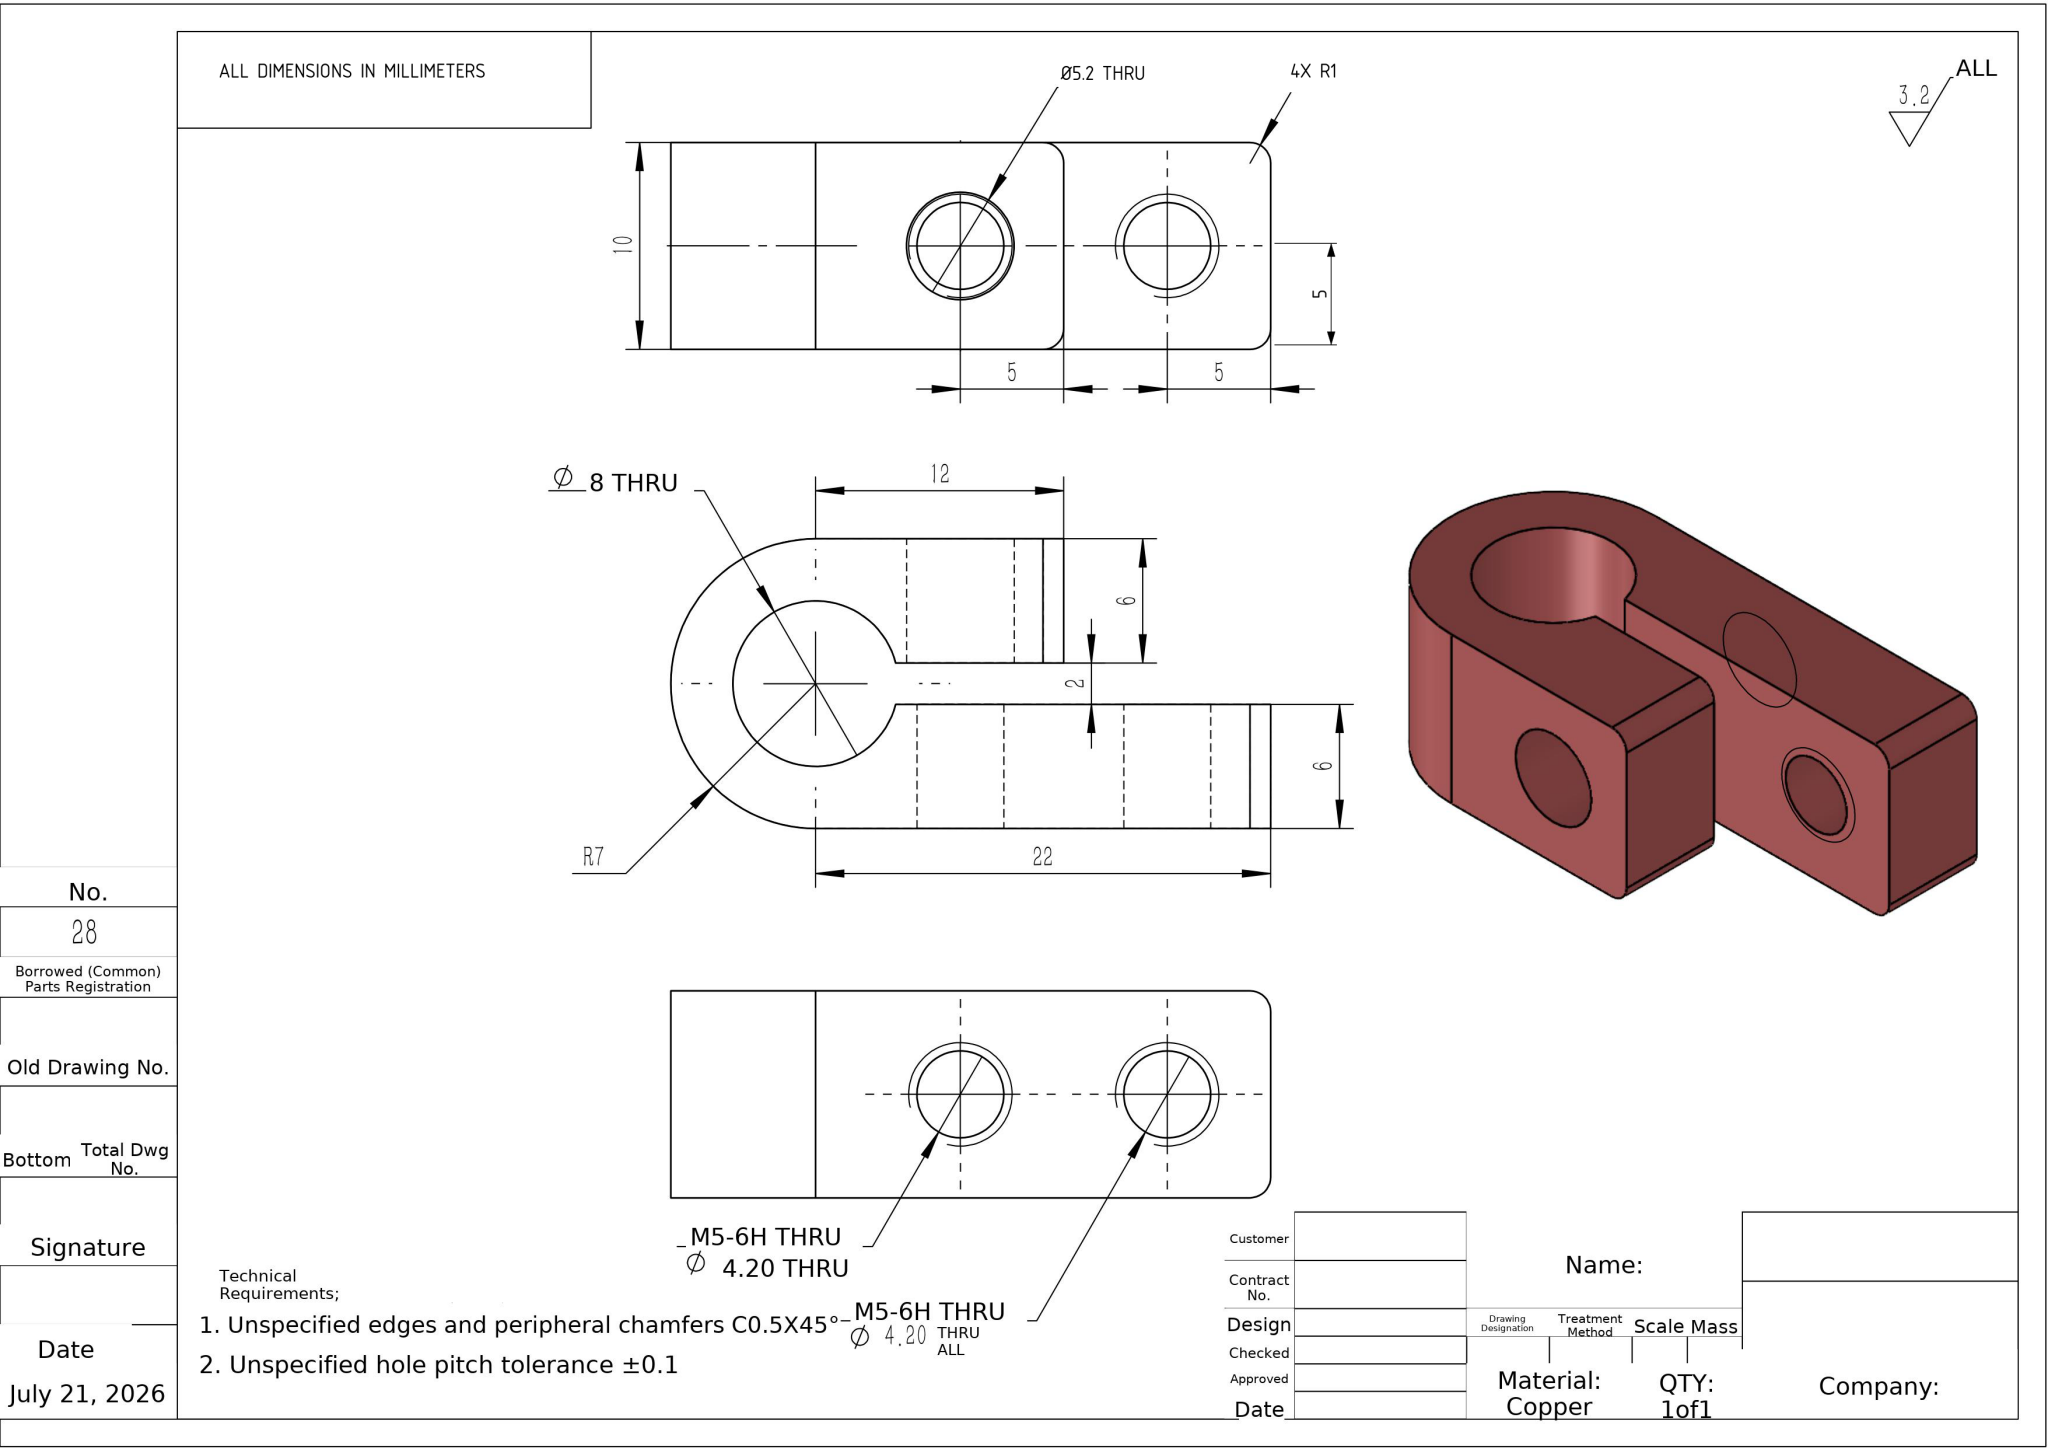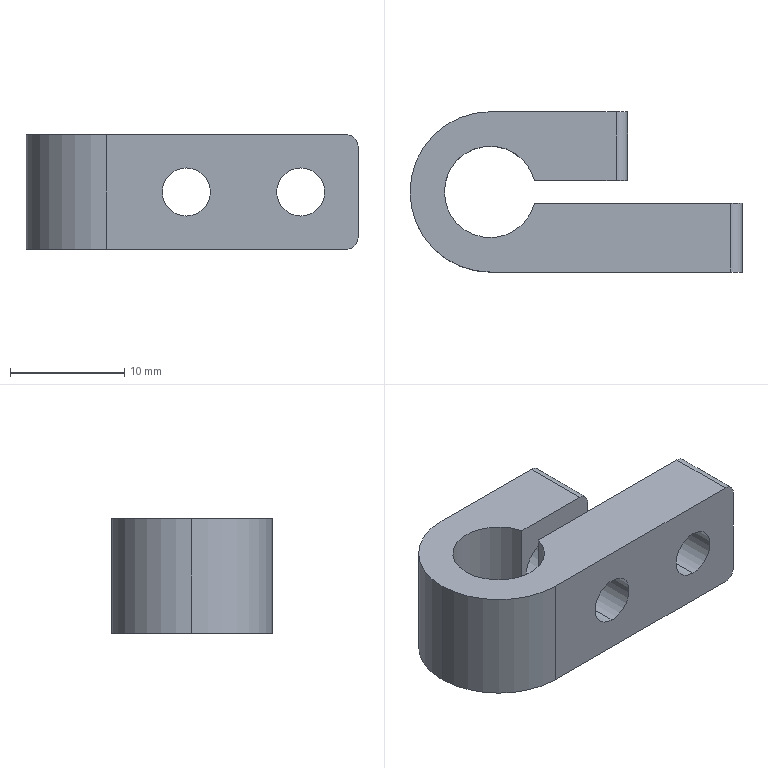Part | NX | mm | Stepped Clevis Bracket | 1 solid | 21 faces | box 29 x 14 x 10 mm | volume 2087 mm3 | cylinder 13 | plane 8 | commonest cylinder face diameters 4.2 x4 2 x4 5.2 x2 14 x2 8 x1
STEP:
#1=COLOUR_RGB('',0.7922,0.8196,0.9333);
#2=FILL_AREA_STYLE_COLOUR('',#1);
#3=FILL_AREA_STYLE('',(#2));
#4=SURFACE_STYLE_FILL_AREA(#3);
#5=SURFACE_SIDE_STYLE('',(#4));
#6=SURFACE_STYLE_USAGE(.BOTH.,#5);
#7=PRESENTATION_STYLE_ASSIGNMENT((#6));
#8=CARTESIAN_POINT('',(-4.,-1.,7.1));
#9=VERTEX_POINT('',#8);
#10=CARTESIAN_POINT('',(-4.,-1.,2.9));
#11=VERTEX_POINT('',#10);
#12=CARTESIAN_POINT('',(-4.,-1.,5.));
#13=DIRECTION('',(0.,-1.,0.));
#14=DIRECTION('',(1.,0.,0.));
#15=AXIS2_PLACEMENT_3D('',#12,#13,#14);
#16=CIRCLE('',#15,2.1);
#17=EDGE_CURVE('',#9,#11,#16,.T.);
#18=ORIENTED_EDGE('',*,*,#17,.F.);
#19=CARTESIAN_POINT('',(-4.,-7.,7.1));
#20=VERTEX_POINT('',#19);
#21=CARTESIAN_POINT('',(-4.,-7.,7.1));
#22=DIRECTION('',(0.,-1.,0.));
#23=VECTOR('',#22,1000.);
#24=LINE('',#21,#23);
#25=EDGE_CURVE('',#9,#20,#24,.T.);
#26=ORIENTED_EDGE('',*,*,#25,.T.);
#27=CARTESIAN_POINT('',(-4.,-7.,2.9));
#28=VERTEX_POINT('',#27);
#29=CARTESIAN_POINT('',(-4.,-7.,5.));
#30=DIRECTION('',(0.,-1.,0.));
#31=DIRECTION('',(0.,0.,-1.));
#32=AXIS2_PLACEMENT_3D('',#29,#30,#31);
#33=CIRCLE('',#32,2.1);
#34=EDGE_CURVE('',#20,#28,#33,.T.);
#35=ORIENTED_EDGE('',*,*,#34,.T.);
#36=CARTESIAN_POINT('',(-4.,-7.,2.9));
#37=DIRECTION('',(0.,-1.,0.));
#38=VECTOR('',#37,1000.);
#39=LINE('',#36,#38);
#40=EDGE_CURVE('',#11,#28,#39,.T.);
#41=ORIENTED_EDGE('',*,*,#40,.F.);
#42=EDGE_LOOP('',(#18,#26,#35,#41));
#43=FACE_OUTER_BOUND('',#42,.T.);
#44=CARTESIAN_POINT('',(-4.,-7.,5.));
#45=DIRECTION('',(0.,-1.,0.));
#46=DIRECTION('',(0.,0.,-1.));
#47=AXIS2_PLACEMENT_3D('',#44,#45,#46);
#48=CYLINDRICAL_SURFACE('',#47,2.1);
#49=ADVANCED_FACE('',(#43),#48,.F.);
#50=CARTESIAN_POINT('',(-4.,1.,2.4));
#51=VERTEX_POINT('',#50);
#52=CARTESIAN_POINT('',(-4.,1.,7.6));
#53=VERTEX_POINT('',#52);
#54=CARTESIAN_POINT('',(-4.,1.,5.));
#55=DIRECTION('',(-0.,1.,0.));
#56=DIRECTION('',(-1.,-0.,0.));
#57=AXIS2_PLACEMENT_3D('',#54,#55,#56);
#58=CIRCLE('',#57,2.6);
#59=EDGE_CURVE('',#51,#53,#58,.T.);
#60=ORIENTED_EDGE('',*,*,#59,.F.);
#61=CARTESIAN_POINT('',(-4.,7.,2.4));
#62=VERTEX_POINT('',#61);
#63=CARTESIAN_POINT('',(-4.,7.,2.4));
#64=DIRECTION('',(0.,1.,0.));
#65=VECTOR('',#64,1000.);
#66=LINE('',#63,#65);
#67=EDGE_CURVE('',#51,#62,#66,.T.);
#68=ORIENTED_EDGE('',*,*,#67,.T.);
#69=CARTESIAN_POINT('',(-4.,7.,7.6));
#70=VERTEX_POINT('',#69);
#71=CARTESIAN_POINT('',(-4.,7.,5.));
#72=DIRECTION('',(0.,1.,0.));
#73=DIRECTION('',(0.,0.,1.));
#74=AXIS2_PLACEMENT_3D('',#71,#72,#73);
#75=CIRCLE('',#74,2.6);
#76=EDGE_CURVE('',#62,#70,#75,.T.);
#77=ORIENTED_EDGE('',*,*,#76,.T.);
#78=CARTESIAN_POINT('',(-4.,7.,7.6));
#79=DIRECTION('',(0.,1.,0.));
#80=VECTOR('',#79,1000.);
#81=LINE('',#78,#80);
#82=EDGE_CURVE('',#53,#70,#81,.T.);
#83=ORIENTED_EDGE('',*,*,#82,.F.);
#84=EDGE_LOOP('',(#60,#68,#77,#83));
#85=FACE_OUTER_BOUND('',#84,.T.);
#86=CARTESIAN_POINT('',(-4.,7.,5.));
#87=DIRECTION('',(0.,1.,0.));
#88=DIRECTION('',(0.,0.,1.));
#89=AXIS2_PLACEMENT_3D('',#86,#87,#88);
#90=CYLINDRICAL_SURFACE('',#89,2.6);
#91=ADVANCED_FACE('',(#85),#90,.F.);
#92=CARTESIAN_POINT('',(6.,-7.,2.9));
#93=VERTEX_POINT('',#92);
#94=CARTESIAN_POINT('',(6.,-7.,7.1));
#95=VERTEX_POINT('',#94);
#96=CARTESIAN_POINT('',(6.,-7.,5.));
#97=DIRECTION('',(0.,1.,0.));
#98=DIRECTION('',(0.,0.,1.));
#99=AXIS2_PLACEMENT_3D('',#96,#97,#98);
#100=CIRCLE('',#99,2.1);
#101=EDGE_CURVE('',#93,#95,#100,.T.);
#102=ORIENTED_EDGE('',*,*,#101,.F.);
#103=CARTESIAN_POINT('',(6.,-1.,2.9));
#104=VERTEX_POINT('',#103);
#105=CARTESIAN_POINT('',(6.,-1.,2.9));
#106=DIRECTION('',(0.,1.,0.));
#107=VECTOR('',#106,1000.);
#108=LINE('',#105,#107);
#109=EDGE_CURVE('',#93,#104,#108,.T.);
#110=ORIENTED_EDGE('',*,*,#109,.T.);
#111=CARTESIAN_POINT('',(6.,-1.,7.1));
#112=VERTEX_POINT('',#111);
#113=CARTESIAN_POINT('',(6.,-1.,5.));
#114=DIRECTION('',(0.,1.,0.));
#115=DIRECTION('',(0.,0.,1.));
#116=AXIS2_PLACEMENT_3D('',#113,#114,#115);
#117=CIRCLE('',#116,2.1);
#118=EDGE_CURVE('',#104,#112,#117,.T.);
#119=ORIENTED_EDGE('',*,*,#118,.T.);
#120=CARTESIAN_POINT('',(6.,-1.,7.1));
#121=DIRECTION('',(0.,1.,0.));
#122=VECTOR('',#121,1000.);
#123=LINE('',#120,#122);
#124=EDGE_CURVE('',#95,#112,#123,.T.);
#125=ORIENTED_EDGE('',*,*,#124,.F.);
#126=EDGE_LOOP('',(#102,#110,#119,#125));
#127=FACE_OUTER_BOUND('',#126,.T.);
#128=CARTESIAN_POINT('',(6.,-1.,5.));
#129=DIRECTION('',(0.,1.,0.));
#130=DIRECTION('',(0.,0.,1.));
#131=AXIS2_PLACEMENT_3D('',#128,#129,#130);
#132=CYLINDRICAL_SURFACE('',#131,2.1);
#133=ADVANCED_FACE('',(#127),#132,.F.);
#134=CARTESIAN_POINT('',(-18.,-0.,10.));
#135=VERTEX_POINT('',#134);
#136=CARTESIAN_POINT('',(-11.,-7.,10.));
#137=VERTEX_POINT('',#136);
#138=CARTESIAN_POINT('',(-11.,-0.,10.));
#139=DIRECTION('',(0.,0.,1.));
#140=DIRECTION('',(1.,0.,0.));
#141=AXIS2_PLACEMENT_3D('',#138,#139,#140);
#142=CIRCLE('',#141,7.);
#143=EDGE_CURVE('',#135,#137,#142,.T.);
#144=ORIENTED_EDGE('',*,*,#143,.F.);
#145=CARTESIAN_POINT('',(-18.,-0.,0.));
#146=VERTEX_POINT('',#145);
#147=CARTESIAN_POINT('',(-18.,-0.,10.));
#148=DIRECTION('',(0.,0.,-1.));
#149=VECTOR('',#148,1000.);
#150=LINE('',#147,#149);
#151=EDGE_CURVE('',#135,#146,#150,.T.);
#152=ORIENTED_EDGE('',*,*,#151,.T.);
#153=CARTESIAN_POINT('',(-11.,-7.,0.));
#154=VERTEX_POINT('',#153);
#155=CARTESIAN_POINT('',(-11.,-0.,0.));
#156=DIRECTION('',(0.,0.,1.));
#157=DIRECTION('',(1.,0.,0.));
#158=AXIS2_PLACEMENT_3D('',#155,#156,#157);
#159=CIRCLE('',#158,7.);
#160=EDGE_CURVE('',#146,#154,#159,.T.);
#161=ORIENTED_EDGE('',*,*,#160,.T.);
#162=CARTESIAN_POINT('',(-11.,-7.,10.));
#163=DIRECTION('',(0.,0.,-1.));
#164=VECTOR('',#163,1000.);
#165=LINE('',#162,#164);
#166=EDGE_CURVE('',#137,#154,#165,.T.);
#167=ORIENTED_EDGE('',*,*,#166,.F.);
#168=EDGE_LOOP('',(#144,#152,#161,#167));
#169=FACE_OUTER_BOUND('',#168,.T.);
#170=CARTESIAN_POINT('',(-11.,-0.,10.));
#171=DIRECTION('',(0.,0.,-1.));
#172=DIRECTION('',(-1.,0.,0.));
#173=AXIS2_PLACEMENT_3D('',#170,#171,#172);
#174=CYLINDRICAL_SURFACE('',#173,7.);
#175=ADVANCED_FACE('',(#169),#174,.T.);
#176=CARTESIAN_POINT('',(-4.,-7.,5.));
#177=DIRECTION('',(0.,-1.,0.));
#178=DIRECTION('',(0.,0.,-1.));
#179=AXIS2_PLACEMENT_3D('',#176,#177,#178);
#180=CIRCLE('',#179,2.1);
#181=EDGE_CURVE('',#28,#20,#180,.T.);
#182=ORIENTED_EDGE('',*,*,#181,.F.);
#183=ORIENTED_EDGE('',*,*,#34,.F.);
#184=EDGE_LOOP('',(#182,#183));
#185=FACE_BOUND('',#184,.T.);
#186=CARTESIAN_POINT('',(6.,-7.,5.));
#187=DIRECTION('',(0.,1.,0.));
#188=DIRECTION('',(0.,0.,1.));
#189=AXIS2_PLACEMENT_3D('',#186,#187,#188);
#190=CIRCLE('',#189,2.1);
#191=EDGE_CURVE('',#95,#93,#190,.T.);
#192=ORIENTED_EDGE('',*,*,#191,.T.);
#193=ORIENTED_EDGE('',*,*,#101,.T.);
#194=EDGE_LOOP('',(#192,#193));
#195=FACE_BOUND('',#194,.T.);
#196=CARTESIAN_POINT('',(10.,-7.,0.));
#197=VERTEX_POINT('',#196);
#198=CARTESIAN_POINT('',(-11.,-7.,0.));
#199=DIRECTION('',(1.,0.,0.));
#200=VECTOR('',#199,1000.);
#201=LINE('',#198,#200);
#202=EDGE_CURVE('',#154,#197,#201,.T.);
#203=ORIENTED_EDGE('',*,*,#202,.T.);
#204=CARTESIAN_POINT('',(11.,-7.,1.));
#205=VERTEX_POINT('',#204);
#206=CARTESIAN_POINT('',(10.,-7.,1.));
#207=DIRECTION('',(0.,-1.,0.));
#208=DIRECTION('',(0.,0.,1.));
#209=AXIS2_PLACEMENT_3D('',#206,#207,#208);
#210=CIRCLE('',#209,1.);
#211=EDGE_CURVE('',#197,#205,#210,.T.);
#212=ORIENTED_EDGE('',*,*,#211,.T.);
#213=CARTESIAN_POINT('',(11.,-7.,9.));
#214=VERTEX_POINT('',#213);
#215=CARTESIAN_POINT('',(11.,-7.,10.));
#216=DIRECTION('',(0.,0.,-1.));
#217=VECTOR('',#216,1000.);
#218=LINE('',#215,#217);
#219=EDGE_CURVE('',#214,#205,#218,.T.);
#220=ORIENTED_EDGE('',*,*,#219,.F.);
#221=CARTESIAN_POINT('',(10.,-7.,10.));
#222=VERTEX_POINT('',#221);
#223=CARTESIAN_POINT('',(10.,-7.,9.));
#224=DIRECTION('',(0.,-1.,0.));
#225=DIRECTION('',(0.,0.,1.));
#226=AXIS2_PLACEMENT_3D('',#223,#224,#225);
#227=CIRCLE('',#226,1.);
#228=EDGE_CURVE('',#214,#222,#227,.T.);
#229=ORIENTED_EDGE('',*,*,#228,.T.);
#230=CARTESIAN_POINT('',(-11.,-7.,10.));
#231=DIRECTION('',(1.,0.,0.));
#232=VECTOR('',#231,1000.);
#233=LINE('',#230,#232);
#234=EDGE_CURVE('',#137,#222,#233,.T.);
#235=ORIENTED_EDGE('',*,*,#234,.F.);
#236=ORIENTED_EDGE('',*,*,#166,.T.);
#237=EDGE_LOOP('',(#203,#212,#220,#229,#235,#236));
#238=FACE_OUTER_BOUND('',#237,.T.);
#239=CARTESIAN_POINT('',(-11.,-7.,10.));
#240=DIRECTION('',(0.,1.,0.));
#241=DIRECTION('',(0.,0.,1.));
#242=AXIS2_PLACEMENT_3D('',#239,#240,#241);
#243=PLANE('',#242);
#244=ADVANCED_FACE('',(#185,#195,#238),#243,.F.);
#245=ORIENTED_EDGE('',*,*,#219,.T.);
#246=CARTESIAN_POINT('',(11.,-1.,1.));
#247=VERTEX_POINT('',#246);
#248=CARTESIAN_POINT('',(11.,-7.,1.));
#249=DIRECTION('',(0.,1.,0.));
#250=VECTOR('',#249,1000.);
#251=LINE('',#248,#250);
#252=EDGE_CURVE('',#205,#247,#251,.T.);
#253=ORIENTED_EDGE('',*,*,#252,.T.);
#254=CARTESIAN_POINT('',(11.,-1.,9.));
#255=VERTEX_POINT('',#254);
#256=CARTESIAN_POINT('',(11.,-1.,10.));
#257=DIRECTION('',(0.,0.,-1.));
#258=VECTOR('',#257,1000.);
#259=LINE('',#256,#258);
#260=EDGE_CURVE('',#255,#247,#259,.T.);
#261=ORIENTED_EDGE('',*,*,#260,.F.);
#262=CARTESIAN_POINT('',(11.,-7.,9.));
#263=DIRECTION('',(0.,-1.,0.));
#264=VECTOR('',#263,1000.);
#265=LINE('',#262,#264);
#266=EDGE_CURVE('',#255,#214,#265,.T.);
#267=ORIENTED_EDGE('',*,*,#266,.T.);
#268=EDGE_LOOP('',(#245,#253,#261,#267));
#269=FACE_OUTER_BOUND('',#268,.T.);
#270=CARTESIAN_POINT('',(11.,-7.,10.));
#271=DIRECTION('',(-1.,0.,0.));
#272=DIRECTION('',(0.,0.,1.));
#273=AXIS2_PLACEMENT_3D('',#270,#271,#272);
#274=PLANE('',#273);
#275=ADVANCED_FACE('',(#269),#274,.F.);
#276=CARTESIAN_POINT('',(-4.,-1.,5.));
#277=DIRECTION('',(0.,-1.,0.));
#278=DIRECTION('',(1.,0.,0.));
#279=AXIS2_PLACEMENT_3D('',#276,#277,#278);
#280=CIRCLE('',#279,2.1);
#281=EDGE_CURVE('',#11,#9,#280,.T.);
#282=ORIENTED_EDGE('',*,*,#281,.T.);
#283=ORIENTED_EDGE('',*,*,#17,.T.);
#284=EDGE_LOOP('',(#282,#283));
#285=FACE_BOUND('',#284,.T.);
#286=CARTESIAN_POINT('',(6.,-1.,5.));
#287=DIRECTION('',(0.,1.,0.));
#288=DIRECTION('',(0.,0.,1.));
#289=AXIS2_PLACEMENT_3D('',#286,#287,#288);
#290=CIRCLE('',#289,2.1);
#291=EDGE_CURVE('',#112,#104,#290,.T.);
#292=ORIENTED_EDGE('',*,*,#291,.F.);
#293=ORIENTED_EDGE('',*,*,#118,.F.);
#294=EDGE_LOOP('',(#292,#293));
#295=FACE_BOUND('',#294,.T.);
#296=ORIENTED_EDGE('',*,*,#260,.T.);
#297=CARTESIAN_POINT('',(10.,-1.,0.));
#298=VERTEX_POINT('',#297);
#299=CARTESIAN_POINT('',(10.,-1.,1.));
#300=DIRECTION('',(-0.,1.,0.));
#301=DIRECTION('',(1.,0.,0.));
#302=AXIS2_PLACEMENT_3D('',#299,#300,#301);
#303=CIRCLE('',#302,1.);
#304=EDGE_CURVE('',#247,#298,#303,.T.);
#305=ORIENTED_EDGE('',*,*,#304,.T.);
#306=CARTESIAN_POINT('',(-7.127,-1.,0.));
#307=VERTEX_POINT('',#306);
#308=CARTESIAN_POINT('',(11.,-1.,0.));
#309=DIRECTION('',(-1.,-0.,0.));
#310=VECTOR('',#309,1000.);
#311=LINE('',#308,#310);
#312=EDGE_CURVE('',#298,#307,#311,.T.);
#313=ORIENTED_EDGE('',*,*,#312,.T.);
#314=CARTESIAN_POINT('',(-7.127,-1.,10.));
#315=VERTEX_POINT('',#314);
#316=CARTESIAN_POINT('',(-7.127,-1.,10.));
#317=DIRECTION('',(0.,0.,1.));
#318=VECTOR('',#317,1000.);
#319=LINE('',#316,#318);
#320=EDGE_CURVE('',#307,#315,#319,.T.);
#321=ORIENTED_EDGE('',*,*,#320,.T.);
#322=CARTESIAN_POINT('',(10.,-1.,10.));
#323=VERTEX_POINT('',#322);
#324=CARTESIAN_POINT('',(11.,-1.,10.));
#325=DIRECTION('',(-1.,-0.,0.));
#326=VECTOR('',#325,1000.);
#327=LINE('',#324,#326);
#328=EDGE_CURVE('',#323,#315,#327,.T.);
#329=ORIENTED_EDGE('',*,*,#328,.F.);
#330=CARTESIAN_POINT('',(10.,-1.,9.));
#331=DIRECTION('',(-0.,1.,0.));
#332=DIRECTION('',(1.,0.,0.));
#333=AXIS2_PLACEMENT_3D('',#330,#331,#332);
#334=CIRCLE('',#333,1.);
#335=EDGE_CURVE('',#323,#255,#334,.T.);
#336=ORIENTED_EDGE('',*,*,#335,.T.);
#337=EDGE_LOOP('',(#296,#305,#313,#321,#329,#336));
#338=FACE_OUTER_BOUND('',#337,.T.);
#339=CARTESIAN_POINT('',(11.,-1.,10.));
#340=DIRECTION('',(0.,-1.,0.));
#341=DIRECTION('',(1.,0.,0.));
#342=AXIS2_PLACEMENT_3D('',#339,#340,#341);
#343=PLANE('',#342);
#344=ADVANCED_FACE('',(#285,#295,#338),#343,.F.);
#345=CARTESIAN_POINT('',(-4.,1.,5.));
#346=DIRECTION('',(-0.,1.,0.));
#347=DIRECTION('',(-1.,-0.,0.));
#348=AXIS2_PLACEMENT_3D('',#345,#346,#347);
#349=CIRCLE('',#348,2.6);
#350=EDGE_CURVE('',#53,#51,#349,.T.);
#351=ORIENTED_EDGE('',*,*,#350,.T.);
#352=ORIENTED_EDGE('',*,*,#59,.T.);
#353=EDGE_LOOP('',(#351,#352));
#354=FACE_BOUND('',#353,.T.);
#355=CARTESIAN_POINT('',(-7.127,1.,0.));
#356=VERTEX_POINT('',#355);
#357=CARTESIAN_POINT('',(0.,1.,0.));
#358=VERTEX_POINT('',#357);
#359=CARTESIAN_POINT('',(1.,1.,0.));
#360=DIRECTION('',(1.,0.,0.));
#361=VECTOR('',#360,1000.);
#362=LINE('',#359,#361);
#363=EDGE_CURVE('',#356,#358,#362,.T.);
#364=ORIENTED_EDGE('',*,*,#363,.T.);
#365=CARTESIAN_POINT('',(1.,1.,1.));
#366=VERTEX_POINT('',#365);
#367=CARTESIAN_POINT('',(0.,1.,1.));
#368=DIRECTION('',(0.,-1.,0.));
#369=DIRECTION('',(-1.,0.,0.));
#370=AXIS2_PLACEMENT_3D('',#367,#368,#369);
#371=CIRCLE('',#370,1.);
#372=EDGE_CURVE('',#358,#366,#371,.T.);
#373=ORIENTED_EDGE('',*,*,#372,.T.);
#374=CARTESIAN_POINT('',(1.,1.,9.));
#375=VERTEX_POINT('',#374);
#376=CARTESIAN_POINT('',(1.,1.,10.));
#377=DIRECTION('',(0.,0.,-1.));
#378=VECTOR('',#377,1000.);
#379=LINE('',#376,#378);
#380=EDGE_CURVE('',#375,#366,#379,.T.);
#381=ORIENTED_EDGE('',*,*,#380,.F.);
#382=CARTESIAN_POINT('',(0.,1.,10.));
#383=VERTEX_POINT('',#382);
#384=CARTESIAN_POINT('',(0.,1.,9.));
#385=DIRECTION('',(0.,-1.,0.));
#386=DIRECTION('',(-1.,0.,0.));
#387=AXIS2_PLACEMENT_3D('',#384,#385,#386);
#388=CIRCLE('',#387,1.);
#389=EDGE_CURVE('',#375,#383,#388,.T.);
#390=ORIENTED_EDGE('',*,*,#389,.T.);
#391=CARTESIAN_POINT('',(-7.127,1.,10.));
#392=VERTEX_POINT('',#391);
#393=CARTESIAN_POINT('',(1.,1.,10.));
#394=DIRECTION('',(1.,0.,0.));
#395=VECTOR('',#394,1000.);
#396=LINE('',#393,#395);
#397=EDGE_CURVE('',#392,#383,#396,.T.);
#398=ORIENTED_EDGE('',*,*,#397,.F.);
#399=CARTESIAN_POINT('',(-7.127,1.,10.));
#400=DIRECTION('',(0.,0.,-1.));
#401=VECTOR('',#400,1000.);
#402=LINE('',#399,#401);
#403=EDGE_CURVE('',#392,#356,#402,.T.);
#404=ORIENTED_EDGE('',*,*,#403,.T.);
#405=EDGE_LOOP('',(#364,#373,#381,#390,#398,#404));
#406=FACE_OUTER_BOUND('',#405,.T.);
#407=CARTESIAN_POINT('',(1.,1.,10.));
#408=DIRECTION('',(-0.,1.,0.));
#409=DIRECTION('',(-1.,-0.,0.));
#410=AXIS2_PLACEMENT_3D('',#407,#408,#409);
#411=PLANE('',#410);
#412=ADVANCED_FACE('',(#354,#406),#411,.F.);
#413=ORIENTED_EDGE('',*,*,#380,.T.);
#414=CARTESIAN_POINT('',(1.,7.,1.));
#415=VERTEX_POINT('',#414);
#416=CARTESIAN_POINT('',(1.,7.,1.));
#417=DIRECTION('',(-0.,1.,0.));
#418=VECTOR('',#417,1000.);
#419=LINE('',#416,#418);
#420=EDGE_CURVE('',#366,#415,#419,.T.);
#421=ORIENTED_EDGE('',*,*,#420,.T.);
#422=CARTESIAN_POINT('',(1.,7.,9.));
#423=VERTEX_POINT('',#422);
#424=CARTESIAN_POINT('',(1.,7.,10.));
#425=DIRECTION('',(0.,0.,-1.));
#426=VECTOR('',#425,1000.);
#427=LINE('',#424,#426);
#428=EDGE_CURVE('',#423,#415,#427,.T.);
#429=ORIENTED_EDGE('',*,*,#428,.F.);
#430=CARTESIAN_POINT('',(1.,1.,9.));
#431=DIRECTION('',(0.,-1.,0.));
#432=VECTOR('',#431,1000.);
#433=LINE('',#430,#432);
#434=EDGE_CURVE('',#423,#375,#433,.T.);
#435=ORIENTED_EDGE('',*,*,#434,.T.);
#436=EDGE_LOOP('',(#413,#421,#429,#435));
#437=FACE_OUTER_BOUND('',#436,.T.);
#438=CARTESIAN_POINT('',(1.,7.,10.));
#439=DIRECTION('',(-1.,-0.,0.));
#440=DIRECTION('',(0.,-1.,0.));
#441=AXIS2_PLACEMENT_3D('',#438,#439,#440);
#442=PLANE('',#441);
#443=ADVANCED_FACE('',(#437),#442,.F.);
#444=CARTESIAN_POINT('',(-4.,7.,5.));
#445=DIRECTION('',(0.,1.,0.));
#446=DIRECTION('',(0.,0.,1.));
#447=AXIS2_PLACEMENT_3D('',#444,#445,#446);
#448=CIRCLE('',#447,2.6);
#449=EDGE_CURVE('',#70,#62,#448,.T.);
#450=ORIENTED_EDGE('',*,*,#449,.F.);
#451=ORIENTED_EDGE('',*,*,#76,.F.);
#452=EDGE_LOOP('',(#450,#451));
#453=FACE_BOUND('',#452,.T.);
#454=ORIENTED_EDGE('',*,*,#428,.T.);
#455=CARTESIAN_POINT('',(0.,7.,0.));
#456=VERTEX_POINT('',#455);
#457=CARTESIAN_POINT('',(0.,7.,1.));
#458=DIRECTION('',(0.,1.,0.));
#459=DIRECTION('',(0.,0.,-1.));
#460=AXIS2_PLACEMENT_3D('',#457,#458,#459);
#461=CIRCLE('',#460,1.);
#462=EDGE_CURVE('',#415,#456,#461,.T.);
#463=ORIENTED_EDGE('',*,*,#462,.T.);
#464=CARTESIAN_POINT('',(-11.,7.,0.));
#465=VERTEX_POINT('',#464);
#466=CARTESIAN_POINT('',(-11.,7.,0.));
#467=DIRECTION('',(-1.,0.,0.));
#468=VECTOR('',#467,1000.);
#469=LINE('',#466,#468);
#470=EDGE_CURVE('',#456,#465,#469,.T.);
#471=ORIENTED_EDGE('',*,*,#470,.T.);
#472=CARTESIAN_POINT('',(-11.,7.,10.));
#473=VERTEX_POINT('',#472);
#474=CARTESIAN_POINT('',(-11.,7.,10.));
#475=DIRECTION('',(0.,0.,-1.));
#476=VECTOR('',#475,1000.);
#477=LINE('',#474,#476);
#478=EDGE_CURVE('',#473,#465,#477,.T.);
#479=ORIENTED_EDGE('',*,*,#478,.F.);
#480=CARTESIAN_POINT('',(0.,7.,10.));
#481=VERTEX_POINT('',#480);
#482=CARTESIAN_POINT('',(-11.,7.,10.));
#483=DIRECTION('',(-1.,0.,0.));
#484=VECTOR('',#483,1000.);
#485=LINE('',#482,#484);
#486=EDGE_CURVE('',#481,#473,#485,.T.);
#487=ORIENTED_EDGE('',*,*,#486,.F.);
#488=CARTESIAN_POINT('',(-0.,7.,9.));
#489=DIRECTION('',(0.,1.,0.));
#490=DIRECTION('',(0.,0.,-1.));
#491=AXIS2_PLACEMENT_3D('',#488,#489,#490);
#492=CIRCLE('',#491,1.);
#493=EDGE_CURVE('',#481,#423,#492,.T.);
#494=ORIENTED_EDGE('',*,*,#493,.T.);
#495=EDGE_LOOP('',(#454,#463,#471,#479,#487,#494));
#496=FACE_OUTER_BOUND('',#495,.T.);
#497=CARTESIAN_POINT('',(-11.,7.,10.));
#498=DIRECTION('',(0.,-1.,0.));
#499=DIRECTION('',(0.,0.,-1.));
#500=AXIS2_PLACEMENT_3D('',#497,#498,#499);
#501=PLANE('',#500);
#502=ADVANCED_FACE('',(#453,#496),#501,.F.);
#503=ORIENTED_EDGE('',*,*,#151,.F.);
#504=CARTESIAN_POINT('',(-11.,-0.,10.));
#505=DIRECTION('',(0.,0.,1.));
#506=DIRECTION('',(1.,0.,0.));
#507=AXIS2_PLACEMENT_3D('',#504,#505,#506);
#508=CIRCLE('',#507,7.);
#509=EDGE_CURVE('',#473,#135,#508,.T.);
#510=ORIENTED_EDGE('',*,*,#509,.F.);
#511=ORIENTED_EDGE('',*,*,#478,.T.);
#512=CARTESIAN_POINT('',(-11.,-0.,0.));
#513=DIRECTION('',(0.,0.,1.));
#514=DIRECTION('',(1.,0.,0.));
#515=AXIS2_PLACEMENT_3D('',#512,#513,#514);
#516=CIRCLE('',#515,7.);
#517=EDGE_CURVE('',#465,#146,#516,.T.);
#518=ORIENTED_EDGE('',*,*,#517,.T.);
#519=EDGE_LOOP('',(#503,#510,#511,#518));
#520=FACE_OUTER_BOUND('',#519,.T.);
#521=CARTESIAN_POINT('',(-11.,-0.,10.));
#522=DIRECTION('',(0.,0.,-1.));
#523=DIRECTION('',(-1.,0.,0.));
#524=AXIS2_PLACEMENT_3D('',#521,#522,#523);
#525=CYLINDRICAL_SURFACE('',#524,7.);
#526=ADVANCED_FACE('',(#520),#525,.T.);
#527=ORIENTED_EDGE('',*,*,#234,.T.);
#528=CARTESIAN_POINT('',(10.,-1.,10.));
#529=DIRECTION('',(0.,1.,0.));
#530=VECTOR('',#529,1000.);
#531=LINE('',#528,#530);
#532=EDGE_CURVE('',#222,#323,#531,.T.);
#533=ORIENTED_EDGE('',*,*,#532,.T.);
#534=ORIENTED_EDGE('',*,*,#328,.T.);
#535=CARTESIAN_POINT('',(-11.,-0.,10.));
#536=DIRECTION('',(0.,0.,1.));
#537=DIRECTION('',(1.,0.,0.));
#538=AXIS2_PLACEMENT_3D('',#535,#536,#537);
#539=CIRCLE('',#538,4.);
#540=EDGE_CURVE('',#392,#315,#539,.T.);
#541=ORIENTED_EDGE('',*,*,#540,.F.);
#542=ORIENTED_EDGE('',*,*,#397,.T.);
#543=CARTESIAN_POINT('',(-0.,7.,10.));
#544=DIRECTION('',(-0.,1.,0.));
#545=VECTOR('',#544,1000.);
#546=LINE('',#543,#545);
#547=EDGE_CURVE('',#383,#481,#546,.T.);
#548=ORIENTED_EDGE('',*,*,#547,.T.);
#549=ORIENTED_EDGE('',*,*,#486,.T.);
#550=ORIENTED_EDGE('',*,*,#509,.T.);
#551=ORIENTED_EDGE('',*,*,#143,.T.);
#552=EDGE_LOOP('',(#527,#533,#534,#541,#542,#548,#549,#550,#551));
#553=FACE_OUTER_BOUND('',#552,.T.);
#554=CARTESIAN_POINT('',(-11.,-0.,10.));
#555=DIRECTION('',(0.,0.,1.));
#556=DIRECTION('',(1.,0.,0.));
#557=AXIS2_PLACEMENT_3D('',#554,#555,#556);
#558=PLANE('',#557);
#559=ADVANCED_FACE('',(#553),#558,.T.);
#560=ORIENTED_EDGE('',*,*,#312,.F.);
#561=CARTESIAN_POINT('',(10.,-0.,0.));
#562=DIRECTION('',(0.,-1.,0.));
#563=VECTOR('',#562,1000.);
#564=LINE('',#561,#563);
#565=EDGE_CURVE('',#298,#197,#564,.T.);
#566=ORIENTED_EDGE('',*,*,#565,.T.);
#567=ORIENTED_EDGE('',*,*,#202,.F.);
#568=ORIENTED_EDGE('',*,*,#160,.F.);
#569=ORIENTED_EDGE('',*,*,#517,.F.);
#570=ORIENTED_EDGE('',*,*,#470,.F.);
#571=CARTESIAN_POINT('',(0.,0.,0.));
#572=DIRECTION('',(0.,-1.,0.));
#573=VECTOR('',#572,1000.);
#574=LINE('',#571,#573);
#575=EDGE_CURVE('',#456,#358,#574,.T.);
#576=ORIENTED_EDGE('',*,*,#575,.T.);
#577=ORIENTED_EDGE('',*,*,#363,.F.);
#578=CARTESIAN_POINT('',(-11.,-0.,0.));
#579=DIRECTION('',(0.,0.,1.));
#580=DIRECTION('',(1.,0.,0.));
#581=AXIS2_PLACEMENT_3D('',#578,#579,#580);
#582=CIRCLE('',#581,4.);
#583=EDGE_CURVE('',#356,#307,#582,.T.);
#584=ORIENTED_EDGE('',*,*,#583,.T.);
#585=EDGE_LOOP('',(#560,#566,#567,#568,#569,#570,#576,#577,#584));
#586=FACE_OUTER_BOUND('',#585,.T.);
#587=CARTESIAN_POINT('',(-11.,-0.,0.));
#588=DIRECTION('',(0.,0.,1.));
#589=DIRECTION('',(1.,0.,0.));
#590=AXIS2_PLACEMENT_3D('',#587,#588,#589);
#591=PLANE('',#590);
#592=ADVANCED_FACE('',(#586),#591,.F.);
#593=ORIENTED_EDGE('',*,*,#583,.F.);
#594=ORIENTED_EDGE('',*,*,#403,.F.);
#595=ORIENTED_EDGE('',*,*,#540,.T.);
#596=ORIENTED_EDGE('',*,*,#320,.F.);
#597=EDGE_LOOP('',(#593,#594,#595,#596));
#598=FACE_OUTER_BOUND('',#597,.T.);
#599=CARTESIAN_POINT('',(-11.,-0.,10.));
#600=DIRECTION('',(0.,0.,1.));
#601=DIRECTION('',(1.,0.,0.));
#602=AXIS2_PLACEMENT_3D('',#599,#600,#601);
#603=CYLINDRICAL_SURFACE('',#602,4.);
#604=ADVANCED_FACE('',(#598),#603,.F.);
#605=ORIENTED_EDGE('',*,*,#109,.F.);
#606=ORIENTED_EDGE('',*,*,#191,.F.);
#607=ORIENTED_EDGE('',*,*,#124,.T.);
#608=ORIENTED_EDGE('',*,*,#291,.T.);
#609=EDGE_LOOP('',(#605,#606,#607,#608));
#610=FACE_OUTER_BOUND('',#609,.T.);
#611=CARTESIAN_POINT('',(6.,-1.,5.));
#612=DIRECTION('',(0.,1.,0.));
#613=DIRECTION('',(0.,0.,1.));
#614=AXIS2_PLACEMENT_3D('',#611,#612,#613);
#615=CYLINDRICAL_SURFACE('',#614,2.1);
#616=ADVANCED_FACE('',(#610),#615,.F.);
#617=ORIENTED_EDGE('',*,*,#67,.F.);
#618=ORIENTED_EDGE('',*,*,#350,.F.);
#619=ORIENTED_EDGE('',*,*,#82,.T.);
#620=ORIENTED_EDGE('',*,*,#449,.T.);
#621=EDGE_LOOP('',(#617,#618,#619,#620));
#622=FACE_OUTER_BOUND('',#621,.T.);
#623=CARTESIAN_POINT('',(-4.,7.,5.));
#624=DIRECTION('',(0.,1.,0.));
#625=DIRECTION('',(0.,0.,1.));
#626=AXIS2_PLACEMENT_3D('',#623,#624,#625);
#627=CYLINDRICAL_SURFACE('',#626,2.6);
#628=ADVANCED_FACE('',(#622),#627,.F.);
#629=ORIENTED_EDGE('',*,*,#25,.F.);
#630=ORIENTED_EDGE('',*,*,#281,.F.);
#631=ORIENTED_EDGE('',*,*,#40,.T.);
#632=ORIENTED_EDGE('',*,*,#181,.T.);
#633=EDGE_LOOP('',(#629,#630,#631,#632));
#634=FACE_OUTER_BOUND('',#633,.T.);
#635=CARTESIAN_POINT('',(-4.,-7.,5.));
#636=DIRECTION('',(0.,-1.,0.));
#637=DIRECTION('',(0.,0.,-1.));
#638=AXIS2_PLACEMENT_3D('',#635,#636,#637);
#639=CYLINDRICAL_SURFACE('',#638,2.1);
#640=ADVANCED_FACE('',(#634),#639,.F.);
#641=ORIENTED_EDGE('',*,*,#211,.F.);
#642=ORIENTED_EDGE('',*,*,#565,.F.);
#643=ORIENTED_EDGE('',*,*,#304,.F.);
#644=ORIENTED_EDGE('',*,*,#252,.F.);
#645=EDGE_LOOP('',(#641,#642,#643,#644));
#646=FACE_OUTER_BOUND('',#645,.T.);
#647=CARTESIAN_POINT('',(10.,-7.,1.));
#648=DIRECTION('',(0.,1.,0.));
#649=DIRECTION('',(0.,0.,1.));
#650=AXIS2_PLACEMENT_3D('',#647,#648,#649);
#651=CYLINDRICAL_SURFACE('',#650,1.);
#652=ADVANCED_FACE('',(#646),#651,.T.);
#653=ORIENTED_EDGE('',*,*,#228,.F.);
#654=ORIENTED_EDGE('',*,*,#266,.F.);
#655=ORIENTED_EDGE('',*,*,#335,.F.);
#656=ORIENTED_EDGE('',*,*,#532,.F.);
#657=EDGE_LOOP('',(#653,#654,#655,#656));
#658=FACE_OUTER_BOUND('',#657,.T.);
#659=CARTESIAN_POINT('',(10.,-0.,9.));
#660=DIRECTION('',(0.,-1.,0.));
#661=DIRECTION('',(0.,0.,-1.));
#662=AXIS2_PLACEMENT_3D('',#659,#660,#661);
#663=CYLINDRICAL_SURFACE('',#662,1.);
#664=ADVANCED_FACE('',(#658),#663,.T.);
#665=ORIENTED_EDGE('',*,*,#372,.F.);
#666=ORIENTED_EDGE('',*,*,#575,.F.);
#667=ORIENTED_EDGE('',*,*,#462,.F.);
#668=ORIENTED_EDGE('',*,*,#420,.F.);
#669=EDGE_LOOP('',(#665,#666,#667,#668));
#670=FACE_OUTER_BOUND('',#669,.T.);
#671=CARTESIAN_POINT('',(0.,7.,1.));
#672=DIRECTION('',(-0.,1.,0.));
#673=DIRECTION('',(-1.,-0.,0.));
#674=AXIS2_PLACEMENT_3D('',#671,#672,#673);
#675=CYLINDRICAL_SURFACE('',#674,1.);
#676=ADVANCED_FACE('',(#670),#675,.T.);
#677=ORIENTED_EDGE('',*,*,#389,.F.);
#678=ORIENTED_EDGE('',*,*,#434,.F.);
#679=ORIENTED_EDGE('',*,*,#493,.F.);
#680=ORIENTED_EDGE('',*,*,#547,.F.);
#681=EDGE_LOOP('',(#677,#678,#679,#680));
#682=FACE_OUTER_BOUND('',#681,.T.);
#683=CARTESIAN_POINT('',(0.,0.,9.));
#684=DIRECTION('',(0.,-1.,0.));
#685=DIRECTION('',(1.,0.,0.));
#686=AXIS2_PLACEMENT_3D('',#683,#684,#685);
#687=CYLINDRICAL_SURFACE('',#686,1.);
#688=ADVANCED_FACE('',(#682),#687,.T.);
#689=CLOSED_SHELL('',(#49,#91,#133,#175,#244,#275,#344,#412,#443,#502,#526,#559,#592,#604,#616,#628,#640,#652,#664,#676,#688));
#690=MANIFOLD_SOLID_BREP('',#689);
#691=STYLED_ITEM('',(#7),#690);
#692=PRESENTATION_LAYER_ASSIGNMENT('','',(#691));
#693=CARTESIAN_POINT('',(0.,0.,0.));
#694=DIRECTION('',(0.,0.,1.));
#695=DIRECTION('',(1.,0.,0.));
#696=AXIS2_PLACEMENT_3D('',#693,#694,#695);
#697=(LENGTH_UNIT()NAMED_UNIT(*)SI_UNIT(.MILLI.,.METRE.));
#698=UNCERTAINTY_MEASURE_WITH_UNIT(LENGTH_MEASURE(0.00001),#697,'','');
#699=(NAMED_UNIT(*)PLANE_ANGLE_UNIT()SI_UNIT($,.RADIAN.));
#700=(NAMED_UNIT(*)SI_UNIT($,.STERADIAN.)SOLID_ANGLE_UNIT());
#701=(GEOMETRIC_REPRESENTATION_CONTEXT(3)GLOBAL_UNCERTAINTY_ASSIGNED_CONTEXT((#698))GLOBAL_UNIT_ASSIGNED_CONTEXT((#697,#699,#700))REPRESENTATION_CONTEXT('',''));
#702=ADVANCED_BREP_SHAPE_REPRESENTATION('',(#690,#696),#701);
#703=(LENGTH_UNIT()NAMED_UNIT(*)SI_UNIT(.MILLI.,.METRE.));
#704=UNCERTAINTY_MEASURE_WITH_UNIT(LENGTH_MEASURE(0.00001),#703,'','');
#705=(NAMED_UNIT(*)PLANE_ANGLE_UNIT()SI_UNIT($,.RADIAN.));
#706=(NAMED_UNIT(*)SI_UNIT($,.STERADIAN.)SOLID_ANGLE_UNIT());
#707=(GEOMETRIC_REPRESENTATION_CONTEXT(3)GLOBAL_UNCERTAINTY_ASSIGNED_CONTEXT((#704))GLOBAL_UNIT_ASSIGNED_CONTEXT((#703,#705,#706))REPRESENTATION_CONTEXT('',''));
#708=MECHANICAL_DESIGN_GEOMETRIC_PRESENTATION_REPRESENTATION('',(#691),#707);